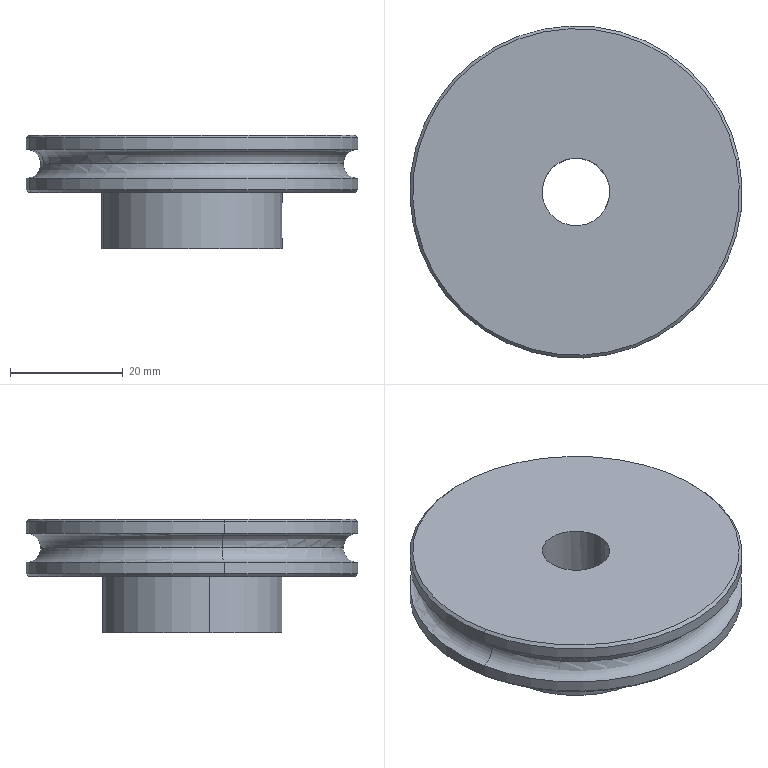Component | SolidWorks | TAR-02-031LargePulley-1 | 1 solid | 21 faces | box 59 x 59 x 20.19 mm | volume 31541 mm3 | cylinder 10 | torus 4 | cone 4 | plane 3 | commonest cylinder face diameters 59 x4 4.2 x2 12 x2 32 x2
build123d program:
from build123d import *

# Parameters (mm, degrees)
SKETCH2_R             = 16
BOSS_EXTRUDE1_DEPTH   = 10
SKETCH3_R             = 6
CUT_EXTRUDE1_DEPTH    = 36
M5_TAPPED_HOLE1_D     = 4.2
M5_TAPPED_HOLE1_DEPTH = 12.4
M5_TAPPED_HOLE1_TIP   = 1.262


with BuildPart() as part:
    # Sketch1 → Revolve1 (revolve)
    with BuildSketch(Plane.XY, mode=Mode.PRIVATE) as revolve1_sk:
        with BuildLine():
            Line((-30.231, 12.507), (-30.231, -16.493))
            Line((-30.231, -16.493), (-20.04, -16.493))
            Line((-20.04, -16.493), (-20.04, 12.507))
            Line((-20.04, 12.507), (-20.54, 13.007))
            Line((-20.54, 13.007), (-22.536, 13.007))
            ThreePointArc((-22.536, 13.007), (-25.136, 10.407), (-27.736, 13.007))
            Line((-27.736, 13.007), (-29.731, 13.007))
            Line((-29.731, 13.007), (-30.231, 12.507))
        make_face()
    revolve(revolve1_sk.sketch.rotate(Axis((-30.231, -16.493, 0), (1, 0, 0)), 90), axis=Axis((-30.231, -16.493, 0), (1, 0, 0)))

    # Sketch2 → Boss-Extrude1 (add)
    with BuildSketch(Plane(origin=(-20.04, 0, 0), x_dir=(0, 0, -1), z_dir=(1, 0, 0))):
        with Locations(Location((0, -16.493, 0), (0, 0, 180))):
            Circle(SKETCH2_R)
    extrude(amount=BOSS_EXTRUDE1_DEPTH)

    # Sketch3 → Cut-Extrude1 (cut)
    with BuildSketch(Plane(origin=(-10.04, 0, 0), x_dir=(0, 0, -1), z_dir=(1, 0, 0))):
        with Locations((0, -16.493)):
            Circle(SKETCH3_R)
    extrude(amount=-CUT_EXTRUDE1_DEPTH, mode=Mode.SUBTRACT)

    # M5 Tapped Hole1
    with Locations(Plane(origin=(-15.04, -16.493, 16), x_dir=(1, 0, 0), z_dir=(0, 0, 1))):
        with Locations((0, 0)):
            Hole(M5_TAPPED_HOLE1_D / 2, depth=M5_TAPPED_HOLE1_DEPTH)
            with Locations((0, 0, -(M5_TAPPED_HOLE1_DEPTH + M5_TAPPED_HOLE1_TIP / 2))):  # 118° drill point
                Cone(0, M5_TAPPED_HOLE1_D / 2, M5_TAPPED_HOLE1_TIP, mode=Mode.SUBTRACT)


solid = part.part

# Placed as in the assembly
solid = solid.moved(Location((11.338, 25.453, -47.696), (-90, 78.561, 90)))
STEP:
#1=CARTESIAN_POINT('',(1.714,0.596,-0.7858));
#2=VERTEX_POINT('',#1);
#3=CARTESIAN_POINT('',(1.613,0.5757,-0.8882));
#4=VERTEX_POINT('',#3);
#5=CARTESIAN_POINT('',(1.714,0.596,-0.8882));
#6=DIRECTION('',(0.1983,-0.9801,0.));
#7=DIRECTION('',(0.9801,0.1983,0.));
#8=AXIS2_PLACEMENT_3D('',#5,#6,#7);
#9=CIRCLE('',#8,0.1024);
#10=EDGE_CURVE('',#2,#4,#9,.T.);
#11=ORIENTED_EDGE('',*,*,#10,.T.);
#12=CARTESIAN_POINT('',(-0.4629,0.1556,-0.8882));
#13=VERTEX_POINT('',#12);
#14=CARTESIAN_POINT('',(0.5752,0.3657,-0.8882));
#15=DIRECTION('',(0.,0.,1.));
#16=DIRECTION('',(1.,0.,0.));
#17=AXIS2_PLACEMENT_3D('',#14,#15,#16);
#18=CIRCLE('',#17,1.059);
#19=EDGE_CURVE('',#4,#13,#18,.T.);
#20=ORIENTED_EDGE('',*,*,#19,.T.);
#21=CARTESIAN_POINT('',(-0.5632,0.1353,-0.7858));
#22=VERTEX_POINT('',#21);
#23=CARTESIAN_POINT('',(-0.5632,0.1353,-0.8882));
#24=DIRECTION('',(-0.1983,0.9801,0.));
#25=DIRECTION('',(-0.9801,-0.1983,0.));
#26=AXIS2_PLACEMENT_3D('',#23,#24,#25);
#27=CIRCLE('',#26,0.1024);
#28=EDGE_CURVE('',#22,#13,#27,.T.);
#29=ORIENTED_EDGE('',*,*,#28,.F.);
#30=CARTESIAN_POINT('',(0.5752,0.3657,-0.7858));
#31=DIRECTION('',(0.,0.,1.));
#32=DIRECTION('',(0.9801,0.1983,0.));
#33=AXIS2_PLACEMENT_3D('',#30,#31,#32);
#34=CIRCLE('',#33,1.161);
#35=EDGE_CURVE('',#2,#22,#34,.T.);
#36=ORIENTED_EDGE('',*,*,#35,.F.);
#37=EDGE_LOOP('',(#11,#20,#29,#36));
#38=FACE_OUTER_BOUND('',#37,.T.);
#39=CARTESIAN_POINT('',(0.5752,0.3657,-0.8882));
#40=DIRECTION('',(0.,0.,1.));
#41=DIRECTION('',(0.9801,0.1983,0.));
#42=AXIS2_PLACEMENT_3D('',#39,#40,#41);
#43=TOROIDAL_SURFACE('',#42,1.161,0.1024);
#44=ADVANCED_FACE('',(#38),#43,.F.);
#45=ORIENTED_EDGE('',*,*,#28,.T.);
#46=CARTESIAN_POINT('',(0.5752,0.3657,-0.8882));
#47=DIRECTION('',(0.,0.,1.));
#48=DIRECTION('',(1.,0.,0.));
#49=AXIS2_PLACEMENT_3D('',#46,#47,#48);
#50=CIRCLE('',#49,1.059);
#51=EDGE_CURVE('',#13,#4,#50,.T.);
#52=ORIENTED_EDGE('',*,*,#51,.T.);
#53=ORIENTED_EDGE('',*,*,#10,.F.);
#54=CARTESIAN_POINT('',(0.5752,0.3657,-0.7858));
#55=DIRECTION('',(0.,0.,1.));
#56=DIRECTION('',(0.9801,0.1983,0.));
#57=AXIS2_PLACEMENT_3D('',#54,#55,#56);
#58=CIRCLE('',#57,1.161);
#59=EDGE_CURVE('',#22,#2,#58,.T.);
#60=ORIENTED_EDGE('',*,*,#59,.F.);
#61=EDGE_LOOP('',(#45,#52,#53,#60));
#62=FACE_OUTER_BOUND('',#61,.T.);
#63=CARTESIAN_POINT('',(0.5752,0.3657,-0.8882));
#64=DIRECTION('',(0.,0.,1.));
#65=DIRECTION('',(0.9801,0.1983,0.));
#66=AXIS2_PLACEMENT_3D('',#63,#64,#65);
#67=TOROIDAL_SURFACE('',#66,1.161,0.1024);
#68=ADVANCED_FACE('',(#62),#67,.F.);
#69=CARTESIAN_POINT('',(0.8067,0.4125,-1.203));
#70=VERTEX_POINT('',#69);
#71=CARTESIAN_POINT('',(0.8067,0.4125,-1.368));
#72=VERTEX_POINT('',#71);
#73=CARTESIAN_POINT('',(0.8067,0.4125,-1.203));
#74=CARTESIAN_POINT('',(0.8078,0.4072,-1.203));
#75=CARTESIAN_POINT('',(0.8087,0.4018,-1.204));
#76=CARTESIAN_POINT('',(0.8101,0.3911,-1.206));
#77=CARTESIAN_POINT('',(0.8106,0.386,-1.207));
#78=CARTESIAN_POINT('',(0.8112,0.3759,-1.211));
#79=CARTESIAN_POINT('',(0.8114,0.371,-1.214));
#80=CARTESIAN_POINT('',(0.8114,0.3619,-1.22));
#81=CARTESIAN_POINT('',(0.8113,0.3577,-1.223));
#82=CARTESIAN_POINT('',(0.8107,0.3459,-1.235));
#83=CARTESIAN_POINT('',(0.81,0.3395,-1.244));
#84=CARTESIAN_POINT('',(0.8091,0.333,-1.259));
#85=CARTESIAN_POINT('',(0.8089,0.3313,-1.264));
#86=CARTESIAN_POINT('',(0.8085,0.3291,-1.275));
#87=CARTESIAN_POINT('',(0.8084,0.3285,-1.28));
#88=CARTESIAN_POINT('',(0.8084,0.3285,-1.291));
#89=CARTESIAN_POINT('',(0.8085,0.3291,-1.297));
#90=CARTESIAN_POINT('',(0.8089,0.3313,-1.307));
#91=CARTESIAN_POINT('',(0.8091,0.333,-1.312));
#92=CARTESIAN_POINT('',(0.81,0.3395,-1.327));
#93=CARTESIAN_POINT('',(0.8107,0.3459,-1.337));
#94=CARTESIAN_POINT('',(0.8113,0.3577,-1.348));
#95=CARTESIAN_POINT('',(0.8114,0.362,-1.351));
#96=CARTESIAN_POINT('',(0.8114,0.3711,-1.357));
#97=CARTESIAN_POINT('',(0.8112,0.3759,-1.36));
#98=CARTESIAN_POINT('',(0.8106,0.386,-1.364));
#99=CARTESIAN_POINT('',(0.8101,0.3912,-1.366));
#100=CARTESIAN_POINT('',(0.8087,0.4018,-1.368));
#101=CARTESIAN_POINT('',(0.8078,0.4071,-1.368));
#102=CARTESIAN_POINT('',(0.8067,0.4125,-1.368));
#103=B_SPLINE_CURVE_WITH_KNOTS('',3,(#73,#74,#75,#76,#77,#78,#79,#80,#81,#82,#83,#84,#85,#86,#87,#88,#89,#90,#91,#92,#93,#94,#95,#96,#97,#98,#99,#100,#101,#102),.UNSPECIFIED.,.F.,.F.,(4,2,2,2,2,2,2,2,2,2,2,2,2,2,4),(0.006618,0.007032,0.007445,0.007859,0.008273,0.0091,0.009513,0.009927,0.01034,0.01075,0.01158,0.01199,0.01241,0.01282,0.01324),.UNSPECIFIED.);
#104=EDGE_CURVE('',#70,#72,#103,.T.);
#105=ORIENTED_EDGE('',*,*,#104,.F.);
#106=CARTESIAN_POINT('',(1.193,0.4906,-1.203));
#107=VERTEX_POINT('',#106);
#108=CARTESIAN_POINT('',(1.193,0.4906,-1.203));
#109=DIRECTION('',(0.9801,0.1983,0.));
#110=VECTOR('',#109,39.37);
#111=LINE('',#108,#110);
#112=EDGE_CURVE('',#70,#107,#111,.T.);
#113=ORIENTED_EDGE('',*,*,#112,.T.);
#114=CARTESIAN_POINT('',(1.193,0.4906,-1.368));
#115=VERTEX_POINT('',#114);
#116=CARTESIAN_POINT('',(1.193,0.4906,-1.368));
#117=CARTESIAN_POINT('',(1.194,0.4852,-1.368));
#118=CARTESIAN_POINT('',(1.195,0.4799,-1.368));
#119=CARTESIAN_POINT('',(1.196,0.4695,-1.366));
#120=CARTESIAN_POINT('',(1.197,0.4643,-1.364));
#121=CARTESIAN_POINT('',(1.199,0.4544,-1.36));
#122=CARTESIAN_POINT('',(1.199,0.4497,-1.357));
#123=CARTESIAN_POINT('',(1.201,0.4408,-1.351));
#124=CARTESIAN_POINT('',(1.201,0.4365,-1.348));
#125=CARTESIAN_POINT('',(1.202,0.4251,-1.336));
#126=CARTESIAN_POINT('',(1.203,0.419,-1.327));
#127=CARTESIAN_POINT('',(1.203,0.4107,-1.307));
#128=CARTESIAN_POINT('',(1.204,0.4085,-1.296));
#129=CARTESIAN_POINT('',(1.204,0.4085,-1.28));
#130=CARTESIAN_POINT('',(1.204,0.409,-1.275));
#131=CARTESIAN_POINT('',(1.203,0.4111,-1.264));
#132=CARTESIAN_POINT('',(1.203,0.4127,-1.259));
#133=CARTESIAN_POINT('',(1.203,0.4169,-1.249));
#134=CARTESIAN_POINT('',(1.203,0.4195,-1.244));
#135=CARTESIAN_POINT('',(1.202,0.4255,-1.235));
#136=CARTESIAN_POINT('',(1.202,0.4289,-1.231));
#137=CARTESIAN_POINT('',(1.201,0.4366,-1.223));
#138=CARTESIAN_POINT('',(1.201,0.4407,-1.22));
#139=CARTESIAN_POINT('',(1.199,0.4497,-1.214));
#140=CARTESIAN_POINT('',(1.199,0.4545,-1.211));
#141=CARTESIAN_POINT('',(1.197,0.4644,-1.207));
#142=CARTESIAN_POINT('',(1.196,0.4695,-1.206));
#143=CARTESIAN_POINT('',(1.195,0.4799,-1.204));
#144=CARTESIAN_POINT('',(1.194,0.4853,-1.203));
#145=CARTESIAN_POINT('',(1.193,0.4906,-1.203));
#146=B_SPLINE_CURVE_WITH_KNOTS('',3,(#116,#117,#118,#119,#120,#121,#122,#123,#124,#125,#126,#127,#128,#129,#130,#131,#132,#133,#134,#135,#136,#137,#138,#139,#140,#141,#142,#143,#144,#145),.UNSPECIFIED.,.F.,.F.,(4,2,2,2,2,2,2,2,2,2,2,2,2,2,4),(0.,0.0004108,0.0008216,0.001232,0.001643,0.002465,0.003286,0.003697,0.004108,0.004519,0.004929,0.00534,0.005751,0.006162,0.006573),.UNSPECIFIED.);
#147=EDGE_CURVE('',#115,#107,#146,.T.);
#148=ORIENTED_EDGE('',*,*,#147,.F.);
#149=CARTESIAN_POINT('',(1.193,0.4906,-1.368));
#150=DIRECTION('',(0.9801,0.1983,0.));
#151=VECTOR('',#150,39.37);
#152=LINE('',#149,#151);
#153=EDGE_CURVE('',#72,#115,#152,.T.);
#154=ORIENTED_EDGE('',*,*,#153,.F.);
#155=EDGE_LOOP('',(#105,#113,#148,#154));
#156=FACE_OUTER_BOUND('',#155,.T.);
#157=CARTESIAN_POINT('',(1.193,0.4906,-1.286));
#158=DIRECTION('',(0.9801,0.1983,0.));
#159=DIRECTION('',(0.,0.,-1.));
#160=AXIS2_PLACEMENT_3D('',#157,#158,#159);
#161=CYLINDRICAL_SURFACE('',#160,0.08268);
#162=ADVANCED_FACE('',(#156),#161,.F.);
#163=CARTESIAN_POINT('',(0.8067,0.4125,-0.6876));
#164=VERTEX_POINT('',#163);
#165=CARTESIAN_POINT('',(0.3436,0.3188,-0.6876));
#166=VERTEX_POINT('',#165);
#167=CARTESIAN_POINT('',(0.5752,0.3657,-0.6876));
#168=DIRECTION('',(0.,0.,-1.));
#169=DIRECTION('',(-0.9801,-0.1983,0.));
#170=AXIS2_PLACEMENT_3D('',#167,#168,#169);
#171=CIRCLE('',#170,0.2362);
#172=EDGE_CURVE('',#164,#166,#171,.T.);
#173=ORIENTED_EDGE('',*,*,#172,.F.);
#174=CARTESIAN_POINT('',(0.8067,0.4125,-0.06517));
#175=DIRECTION('',(0.,0.,-1.));
#176=VECTOR('',#175,39.37);
#177=LINE('',#174,#176);
#178=EDGE_CURVE('',#164,#70,#177,.T.);
#179=ORIENTED_EDGE('',*,*,#178,.T.);
#180=ORIENTED_EDGE('',*,*,#104,.T.);
#181=CARTESIAN_POINT('',(0.8067,0.4125,-1.482));
#182=VERTEX_POINT('',#181);
#183=CARTESIAN_POINT('',(0.8067,0.4125,-0.06517));
#184=DIRECTION('',(0.,0.,-1.));
#185=VECTOR('',#184,39.37);
#186=LINE('',#183,#185);
#187=EDGE_CURVE('',#72,#182,#186,.T.);
#188=ORIENTED_EDGE('',*,*,#187,.T.);
#189=CARTESIAN_POINT('',(0.3436,0.3188,-1.482));
#190=VERTEX_POINT('',#189);
#191=CARTESIAN_POINT('',(0.5752,0.3657,-1.482));
#192=DIRECTION('',(0.,0.,-1.));
#193=DIRECTION('',(-0.9801,-0.1983,0.));
#194=AXIS2_PLACEMENT_3D('',#191,#192,#193);
#195=CIRCLE('',#194,0.2362);
#196=EDGE_CURVE('',#182,#190,#195,.T.);
#197=ORIENTED_EDGE('',*,*,#196,.T.);
#198=CARTESIAN_POINT('',(0.3436,0.3188,-0.06517));
#199=DIRECTION('',(0.,0.,-1.));
#200=VECTOR('',#199,39.37);
#201=LINE('',#198,#200);
#202=EDGE_CURVE('',#166,#190,#201,.T.);
#203=ORIENTED_EDGE('',*,*,#202,.F.);
#204=EDGE_LOOP('',(#173,#179,#180,#188,#197,#203));
#205=FACE_OUTER_BOUND('',#204,.T.);
#206=CARTESIAN_POINT('',(0.5752,0.3657,-0.06517));
#207=DIRECTION('',(0.,0.,-1.));
#208=DIRECTION('',(-0.9801,-0.1983,0.));
#209=AXIS2_PLACEMENT_3D('',#206,#207,#208);
#210=CYLINDRICAL_SURFACE('',#209,0.2362);
#211=ADVANCED_FACE('',(#205),#210,.F.);
#212=CARTESIAN_POINT('',(-0.04225,0.2407,-1.482));
#213=VERTEX_POINT('',#212);
#214=CARTESIAN_POINT('',(1.193,0.4906,-1.482));
#215=VERTEX_POINT('',#214);
#216=CARTESIAN_POINT('',(0.5752,0.3657,-1.482));
#217=DIRECTION('',(0.,0.,-1.));
#218=DIRECTION('',(-0.9801,-0.1983,0.));
#219=AXIS2_PLACEMENT_3D('',#216,#217,#218);
#220=CIRCLE('',#219,0.6299);
#221=EDGE_CURVE('',#213,#215,#220,.T.);
#222=ORIENTED_EDGE('',*,*,#221,.F.);
#223=CARTESIAN_POINT('',(-0.04225,0.2407,-1.089));
#224=VERTEX_POINT('',#223);
#225=CARTESIAN_POINT('',(-0.04225,0.2407,-1.482));
#226=DIRECTION('',(0.,0.,1.));
#227=VECTOR('',#226,39.37);
#228=LINE('',#225,#227);
#229=EDGE_CURVE('',#213,#224,#228,.T.);
#230=ORIENTED_EDGE('',*,*,#229,.T.);
#231=CARTESIAN_POINT('',(1.193,0.4906,-1.089));
#232=VERTEX_POINT('',#231);
#233=CARTESIAN_POINT('',(0.5752,0.3657,-1.089));
#234=DIRECTION('',(0.,0.,-1.));
#235=DIRECTION('',(0.9801,0.1983,0.));
#236=AXIS2_PLACEMENT_3D('',#233,#234,#235);
#237=CIRCLE('',#236,0.6299);
#238=EDGE_CURVE('',#224,#232,#237,.T.);
#239=ORIENTED_EDGE('',*,*,#238,.T.);
#240=CARTESIAN_POINT('',(1.193,0.4906,-1.482));
#241=DIRECTION('',(0.,0.,1.));
#242=VECTOR('',#241,39.37);
#243=LINE('',#240,#242);
#244=EDGE_CURVE('',#107,#232,#243,.T.);
#245=ORIENTED_EDGE('',*,*,#244,.F.);
#246=CARTESIAN_POINT('',(1.193,0.4906,-1.203));
#247=CARTESIAN_POINT('',(1.19,0.5012,-1.203));
#248=CARTESIAN_POINT('',(1.188,0.5118,-1.205));
#249=CARTESIAN_POINT('',(1.183,0.5311,-1.213));
#250=CARTESIAN_POINT('',(1.181,0.54,-1.22));
#251=CARTESIAN_POINT('',(1.177,0.551,-1.231));
#252=CARTESIAN_POINT('',(1.176,0.5543,-1.235));
#253=CARTESIAN_POINT('',(1.174,0.5601,-1.244));
#254=CARTESIAN_POINT('',(1.174,0.5625,-1.249));
#255=CARTESIAN_POINT('',(1.172,0.5665,-1.259));
#256=CARTESIAN_POINT('',(1.172,0.568,-1.264));
#257=CARTESIAN_POINT('',(1.171,0.57,-1.275));
#258=CARTESIAN_POINT('',(1.171,0.5705,-1.28));
#259=CARTESIAN_POINT('',(1.171,0.5705,-1.291));
#260=CARTESIAN_POINT('',(1.171,0.57,-1.296));
#261=CARTESIAN_POINT('',(1.172,0.568,-1.307));
#262=CARTESIAN_POINT('',(1.172,0.5665,-1.312));
#263=CARTESIAN_POINT('',(1.174,0.5626,-1.322));
#264=CARTESIAN_POINT('',(1.174,0.5601,-1.327));
#265=CARTESIAN_POINT('',(1.176,0.5544,-1.336));
#266=CARTESIAN_POINT('',(1.177,0.551,-1.34));
#267=CARTESIAN_POINT('',(1.181,0.5401,-1.352));
#268=CARTESIAN_POINT('',(1.183,0.5312,-1.358));
#269=CARTESIAN_POINT('',(1.188,0.5119,-1.366));
#270=CARTESIAN_POINT('',(1.19,0.5013,-1.368));
#271=CARTESIAN_POINT('',(1.193,0.4906,-1.368));
#272=B_SPLINE_CURVE_WITH_KNOTS('',3,(#246,#247,#248,#249,#250,#251,#252,#253,#254,#255,#256,#257,#258,#259,#260,#261,#262,#263,#264,#265,#266,#267,#268,#269,#270,#271),.UNSPECIFIED.,.F.,.F.,(4,2,2,2,2,2,2,2,2,2,2,2,4),(0.006573,0.007394,0.008215,0.008626,0.009037,0.009447,0.009858,0.01027,0.01068,0.01109,0.0115,0.01232,0.01314),.UNSPECIFIED.);
#273=EDGE_CURVE('',#107,#115,#272,.T.);
#274=ORIENTED_EDGE('',*,*,#273,.T.);
#275=CARTESIAN_POINT('',(1.193,0.4906,-1.482));
#276=DIRECTION('',(0.,0.,1.));
#277=VECTOR('',#276,39.37);
#278=LINE('',#275,#277);
#279=EDGE_CURVE('',#215,#115,#278,.T.);
#280=ORIENTED_EDGE('',*,*,#279,.F.);
#281=EDGE_LOOP('',(#222,#230,#239,#245,#274,#280));
#282=FACE_OUTER_BOUND('',#281,.T.);
#283=CARTESIAN_POINT('',(0.5752,0.3657,-1.482));
#284=DIRECTION('',(0.,0.,1.));
#285=DIRECTION('',(0.9801,0.1983,0.));
#286=AXIS2_PLACEMENT_3D('',#283,#284,#285);
#287=CYLINDRICAL_SURFACE('',#286,0.6299);
#288=ADVANCED_FACE('',(#282),#287,.T.);
#289=CARTESIAN_POINT('',(1.694,0.5921,-0.6876));
#290=VERTEX_POINT('',#289);
#291=CARTESIAN_POINT('',(-0.5439,0.1392,-0.6876));
#292=VERTEX_POINT('',#291);
#293=CARTESIAN_POINT('',(0.5752,0.3657,-0.6876));
#294=DIRECTION('',(0.,0.,1.));
#295=DIRECTION('',(0.9801,0.1983,0.));
#296=AXIS2_PLACEMENT_3D('',#293,#294,#295);
#297=CIRCLE('',#296,1.142);
#298=EDGE_CURVE('',#290,#292,#297,.T.);
#299=ORIENTED_EDGE('',*,*,#298,.F.);
#300=CARTESIAN_POINT('',(1.714,0.596,-0.7073));
#301=VERTEX_POINT('',#300);
#302=CARTESIAN_POINT('',(1.714,0.596,-0.7073));
#303=DIRECTION('',(0.6931,0.1402,-0.7071));
#304=VECTOR('',#303,39.37);
#305=LINE('',#302,#304);
#306=EDGE_CURVE('',#290,#301,#305,.T.);
#307=ORIENTED_EDGE('',*,*,#306,.T.);
#308=CARTESIAN_POINT('',(-0.5632,0.1353,-0.7073));
#309=VERTEX_POINT('',#308);
#310=CARTESIAN_POINT('',(0.5752,0.3657,-0.7073));
#311=DIRECTION('',(0.,0.,1.));
#312=DIRECTION('',(0.9801,0.1983,0.));
#313=AXIS2_PLACEMENT_3D('',#310,#311,#312);
#314=CIRCLE('',#313,1.161);
#315=EDGE_CURVE('',#301,#309,#314,.T.);
#316=ORIENTED_EDGE('',*,*,#315,.T.);
#317=CARTESIAN_POINT('',(-0.5632,0.1353,-0.7073));
#318=DIRECTION('',(-0.6931,-0.1402,-0.7071));
#319=VECTOR('',#318,39.37);
#320=LINE('',#317,#319);
#321=EDGE_CURVE('',#292,#309,#320,.T.);
#322=ORIENTED_EDGE('',*,*,#321,.F.);
#323=EDGE_LOOP('',(#299,#307,#316,#322));
#324=FACE_OUTER_BOUND('',#323,.T.);
#325=CARTESIAN_POINT('',(0.5752,0.3657,-0.7073));
#326=DIRECTION('',(0.,0.,-1.));
#327=DIRECTION('',(-0.9801,-0.1983,0.));
#328=AXIS2_PLACEMENT_3D('',#325,#326,#327);
#329=CONICAL_SURFACE('',#328,1.161,0.7854);
#330=ADVANCED_FACE('',(#324),#329,.T.);
#331=ORIENTED_EDGE('',*,*,#35,.T.);
#332=CARTESIAN_POINT('',(-0.5632,0.1353,-0.6876));
#333=DIRECTION('',(0.,0.,1.));
#334=VECTOR('',#333,39.37);
#335=LINE('',#332,#334);
#336=EDGE_CURVE('',#22,#309,#335,.T.);
#337=ORIENTED_EDGE('',*,*,#336,.T.);
#338=ORIENTED_EDGE('',*,*,#315,.F.);
#339=CARTESIAN_POINT('',(1.714,0.596,-0.6876));
#340=DIRECTION('',(0.,0.,1.));
#341=VECTOR('',#340,39.37);
#342=LINE('',#339,#341);
#343=EDGE_CURVE('',#2,#301,#342,.T.);
#344=ORIENTED_EDGE('',*,*,#343,.F.);
#345=EDGE_LOOP('',(#331,#337,#338,#344));
#346=FACE_OUTER_BOUND('',#345,.T.);
#347=CARTESIAN_POINT('',(0.5752,0.3657,-0.6876));
#348=DIRECTION('',(0.,0.,1.));
#349=DIRECTION('',(0.9801,0.1983,0.));
#350=AXIS2_PLACEMENT_3D('',#347,#348,#349);
#351=CYLINDRICAL_SURFACE('',#350,1.161);
#352=ADVANCED_FACE('',(#346),#351,.T.);
#353=ORIENTED_EDGE('',*,*,#51,.F.);
#354=CARTESIAN_POINT('',(-0.5632,0.1353,-0.9905));
#355=VERTEX_POINT('',#354);
#356=CARTESIAN_POINT('',(-0.5632,0.1353,-0.8882));
#357=DIRECTION('',(-0.1983,0.9801,0.));
#358=DIRECTION('',(-0.9801,-0.1983,0.));
#359=AXIS2_PLACEMENT_3D('',#356,#357,#358);
#360=CIRCLE('',#359,0.1024);
#361=EDGE_CURVE('',#13,#355,#360,.T.);
#362=ORIENTED_EDGE('',*,*,#361,.T.);
#363=CARTESIAN_POINT('',(1.714,0.596,-0.9905));
#364=VERTEX_POINT('',#363);
#365=CARTESIAN_POINT('',(0.5752,0.3657,-0.9905));
#366=DIRECTION('',(0.,0.,1.));
#367=DIRECTION('',(0.9801,0.1983,0.));
#368=AXIS2_PLACEMENT_3D('',#365,#366,#367);
#369=CIRCLE('',#368,1.161);
#370=EDGE_CURVE('',#355,#364,#369,.T.);
#371=ORIENTED_EDGE('',*,*,#370,.T.);
#372=CARTESIAN_POINT('',(1.714,0.596,-0.8882));
#373=DIRECTION('',(0.1983,-0.9801,0.));
#374=DIRECTION('',(0.9801,0.1983,0.));
#375=AXIS2_PLACEMENT_3D('',#372,#373,#374);
#376=CIRCLE('',#375,0.1024);
#377=EDGE_CURVE('',#4,#364,#376,.T.);
#378=ORIENTED_EDGE('',*,*,#377,.F.);
#379=EDGE_LOOP('',(#353,#362,#371,#378));
#380=FACE_OUTER_BOUND('',#379,.T.);
#381=CARTESIAN_POINT('',(0.5752,0.3657,-0.8882));
#382=DIRECTION('',(0.,0.,1.));
#383=DIRECTION('',(0.9801,0.1983,0.));
#384=AXIS2_PLACEMENT_3D('',#381,#382,#383);
#385=TOROIDAL_SURFACE('',#384,1.161,0.1024);
#386=ADVANCED_FACE('',(#380),#385,.F.);
#387=CARTESIAN_POINT('',(1.714,0.596,-1.069));
#388=VERTEX_POINT('',#387);
#389=CARTESIAN_POINT('',(-0.5632,0.1353,-1.069));
#390=VERTEX_POINT('',#389);
#391=CARTESIAN_POINT('',(0.5752,0.3657,-1.069));
#392=DIRECTION('',(0.,0.,1.));
#393=DIRECTION('',(0.9801,0.1983,0.));
#394=AXIS2_PLACEMENT_3D('',#391,#392,#393);
#395=CIRCLE('',#394,1.161);
#396=EDGE_CURVE('',#388,#390,#395,.T.);
#397=ORIENTED_EDGE('',*,*,#396,.T.);
#398=CARTESIAN_POINT('',(-0.5632,0.1353,-0.6876));
#399=DIRECTION('',(0.,0.,1.));
#400=VECTOR('',#399,39.37);
#401=LINE('',#398,#400);
#402=EDGE_CURVE('',#390,#355,#401,.T.);
#403=ORIENTED_EDGE('',*,*,#402,.T.);
#404=CARTESIAN_POINT('',(0.5752,0.3657,-0.9905));
#405=DIRECTION('',(0.,0.,1.));
#406=DIRECTION('',(0.9801,0.1983,0.));
#407=AXIS2_PLACEMENT_3D('',#404,#405,#406);
#408=CIRCLE('',#407,1.161);
#409=EDGE_CURVE('',#364,#355,#408,.T.);
#410=ORIENTED_EDGE('',*,*,#409,.F.);
#411=CARTESIAN_POINT('',(1.714,0.596,-0.6876));
#412=DIRECTION('',(0.,0.,1.));
#413=VECTOR('',#412,39.37);
#414=LINE('',#411,#413);
#415=EDGE_CURVE('',#388,#364,#414,.T.);
#416=ORIENTED_EDGE('',*,*,#415,.F.);
#417=EDGE_LOOP('',(#397,#403,#410,#416));
#418=FACE_OUTER_BOUND('',#417,.T.);
#419=CARTESIAN_POINT('',(0.5752,0.3657,-0.6876));
#420=DIRECTION('',(0.,0.,1.));
#421=DIRECTION('',(0.9801,0.1983,0.));
#422=AXIS2_PLACEMENT_3D('',#419,#420,#421);
#423=CYLINDRICAL_SURFACE('',#422,1.161);
#424=ADVANCED_FACE('',(#418),#423,.T.);
#425=CARTESIAN_POINT('',(1.694,0.5921,-1.089));
#426=VERTEX_POINT('',#425);
#427=CARTESIAN_POINT('',(-0.5439,0.1392,-1.089));
#428=VERTEX_POINT('',#427);
#429=CARTESIAN_POINT('',(0.5752,0.3657,-1.089));
#430=DIRECTION('',(0.,0.,1.));
#431=DIRECTION('',(0.9801,0.1983,0.));
#432=AXIS2_PLACEMENT_3D('',#429,#430,#431);
#433=CIRCLE('',#432,1.142);
#434=EDGE_CURVE('',#426,#428,#433,.T.);
#435=ORIENTED_EDGE('',*,*,#434,.T.);
#436=CARTESIAN_POINT('',(-0.5439,0.1392,-1.089));
#437=DIRECTION('',(-0.6931,-0.1402,0.7071));
#438=VECTOR('',#437,39.37);
#439=LINE('',#436,#438);
#440=EDGE_CURVE('',#428,#390,#439,.T.);
#441=ORIENTED_EDGE('',*,*,#440,.T.);
#442=ORIENTED_EDGE('',*,*,#396,.F.);
#443=CARTESIAN_POINT('',(1.694,0.5921,-1.089));
#444=DIRECTION('',(0.6931,0.1402,0.7071));
#445=VECTOR('',#444,39.37);
#446=LINE('',#443,#445);
#447=EDGE_CURVE('',#426,#388,#446,.T.);
#448=ORIENTED_EDGE('',*,*,#447,.F.);
#449=EDGE_LOOP('',(#435,#441,#442,#448));
#450=FACE_OUTER_BOUND('',#449,.T.);
#451=CARTESIAN_POINT('',(0.5752,0.3657,-1.089));
#452=DIRECTION('',(0.,0.,1.));
#453=DIRECTION('',(0.9801,0.1983,0.));
#454=AXIS2_PLACEMENT_3D('',#451,#452,#453);
#455=CONICAL_SURFACE('',#454,1.142,0.7854);
#456=ADVANCED_FACE('',(#450),#455,.T.);
#457=CARTESIAN_POINT('',(0.5752,0.3657,-1.089));
#458=DIRECTION('',(0.,0.,-1.));
#459=DIRECTION('',(0.9801,0.1983,0.));
#460=AXIS2_PLACEMENT_3D('',#457,#458,#459);
#461=CIRCLE('',#460,0.6299);
#462=EDGE_CURVE('',#232,#224,#461,.T.);
#463=ORIENTED_EDGE('',*,*,#462,.F.);
#464=ORIENTED_EDGE('',*,*,#238,.F.);
#465=EDGE_LOOP('',(#463,#464));
#466=FACE_BOUND('',#465,.T.);
#467=ORIENTED_EDGE('',*,*,#434,.F.);
#468=CARTESIAN_POINT('',(0.5752,0.3657,-1.089));
#469=DIRECTION('',(0.,0.,1.));
#470=DIRECTION('',(0.9801,0.1983,0.));
#471=AXIS2_PLACEMENT_3D('',#468,#469,#470);
#472=CIRCLE('',#471,1.142);
#473=EDGE_CURVE('',#428,#426,#472,.T.);
#474=ORIENTED_EDGE('',*,*,#473,.F.);
#475=EDGE_LOOP('',(#467,#474));
#476=FACE_OUTER_BOUND('',#475,.T.);
#477=CARTESIAN_POINT('',(0.5752,0.3657,-1.089));
#478=DIRECTION('',(0.,0.,1.));
#479=DIRECTION('',(0.9801,0.1983,0.));
#480=AXIS2_PLACEMENT_3D('',#477,#478,#479);
#481=PLANE('',#480);
#482=ADVANCED_FACE('',(#466,#476),#481,.F.);
#483=ORIENTED_EDGE('',*,*,#440,.F.);
#484=ORIENTED_EDGE('',*,*,#473,.T.);
#485=ORIENTED_EDGE('',*,*,#447,.T.);
#486=CARTESIAN_POINT('',(0.5752,0.3657,-1.069));
#487=DIRECTION('',(0.,0.,1.));
#488=DIRECTION('',(0.9801,0.1983,0.));
#489=AXIS2_PLACEMENT_3D('',#486,#487,#488);
#490=CIRCLE('',#489,1.161);
#491=EDGE_CURVE('',#390,#388,#490,.T.);
#492=ORIENTED_EDGE('',*,*,#491,.F.);
#493=EDGE_LOOP('',(#483,#484,#485,#492));
#494=FACE_OUTER_BOUND('',#493,.T.);
#495=CARTESIAN_POINT('',(0.5752,0.3657,-1.089));
#496=DIRECTION('',(0.,0.,1.));
#497=DIRECTION('',(0.9801,0.1983,0.));
#498=AXIS2_PLACEMENT_3D('',#495,#496,#497);
#499=CONICAL_SURFACE('',#498,1.142,0.7854);
#500=ADVANCED_FACE('',(#494),#499,.T.);
#501=ORIENTED_EDGE('',*,*,#402,.F.);
#502=ORIENTED_EDGE('',*,*,#491,.T.);
#503=ORIENTED_EDGE('',*,*,#415,.T.);
#504=ORIENTED_EDGE('',*,*,#370,.F.);
#505=EDGE_LOOP('',(#501,#502,#503,#504));
#506=FACE_OUTER_BOUND('',#505,.T.);
#507=CARTESIAN_POINT('',(0.5752,0.3657,-0.6876));
#508=DIRECTION('',(0.,0.,1.));
#509=DIRECTION('',(0.9801,0.1983,0.));
#510=AXIS2_PLACEMENT_3D('',#507,#508,#509);
#511=CYLINDRICAL_SURFACE('',#510,1.161);
#512=ADVANCED_FACE('',(#506),#511,.T.);
#513=ORIENTED_EDGE('',*,*,#19,.F.);
#514=ORIENTED_EDGE('',*,*,#377,.T.);
#515=ORIENTED_EDGE('',*,*,#409,.T.);
#516=ORIENTED_EDGE('',*,*,#361,.F.);
#517=EDGE_LOOP('',(#513,#514,#515,#516));
#518=FACE_OUTER_BOUND('',#517,.T.);
#519=CARTESIAN_POINT('',(0.5752,0.3657,-0.8882));
#520=DIRECTION('',(0.,0.,1.));
#521=DIRECTION('',(0.9801,0.1983,0.));
#522=AXIS2_PLACEMENT_3D('',#519,#520,#521);
#523=TOROIDAL_SURFACE('',#522,1.161,0.1024);
#524=ADVANCED_FACE('',(#518),#523,.F.);
#525=ORIENTED_EDGE('',*,*,#336,.F.);
#526=ORIENTED_EDGE('',*,*,#59,.T.);
#527=ORIENTED_EDGE('',*,*,#343,.T.);
#528=CARTESIAN_POINT('',(0.5752,0.3657,-0.7073));
#529=DIRECTION('',(0.,0.,1.));
#530=DIRECTION('',(0.9801,0.1983,0.));
#531=AXIS2_PLACEMENT_3D('',#528,#529,#530);
#532=CIRCLE('',#531,1.161);
#533=EDGE_CURVE('',#309,#301,#532,.T.);
#534=ORIENTED_EDGE('',*,*,#533,.F.);
#535=EDGE_LOOP('',(#525,#526,#527,#534));
#536=FACE_OUTER_BOUND('',#535,.T.);
#537=CARTESIAN_POINT('',(0.5752,0.3657,-0.6876));
#538=DIRECTION('',(0.,0.,1.));
#539=DIRECTION('',(0.9801,0.1983,0.));
#540=AXIS2_PLACEMENT_3D('',#537,#538,#539);
#541=CYLINDRICAL_SURFACE('',#540,1.161);
#542=ADVANCED_FACE('',(#536),#541,.T.);
#543=ORIENTED_EDGE('',*,*,#306,.F.);
#544=CARTESIAN_POINT('',(0.5752,0.3657,-0.6876));
#545=DIRECTION('',(0.,0.,1.));
#546=DIRECTION('',(0.9801,0.1983,0.));
#547=AXIS2_PLACEMENT_3D('',#544,#545,#546);
#548=CIRCLE('',#547,1.142);
#549=EDGE_CURVE('',#292,#290,#548,.T.);
#550=ORIENTED_EDGE('',*,*,#549,.F.);
#551=ORIENTED_EDGE('',*,*,#321,.T.);
#552=ORIENTED_EDGE('',*,*,#533,.T.);
#553=EDGE_LOOP('',(#543,#550,#551,#552));
#554=FACE_OUTER_BOUND('',#553,.T.);
#555=CARTESIAN_POINT('',(0.5752,0.3657,-0.7073));
#556=DIRECTION('',(0.,0.,-1.));
#557=DIRECTION('',(-0.9801,-0.1983,0.));
#558=AXIS2_PLACEMENT_3D('',#555,#556,#557);
#559=CONICAL_SURFACE('',#558,1.161,0.7854);
#560=ADVANCED_FACE('',(#554),#559,.T.);
#561=CARTESIAN_POINT('',(0.5752,0.3657,-0.6876));
#562=DIRECTION('',(0.,0.,-1.));
#563=DIRECTION('',(-0.9801,-0.1983,0.));
#564=AXIS2_PLACEMENT_3D('',#561,#562,#563);
#565=CIRCLE('',#564,0.2362);
#566=EDGE_CURVE('',#166,#164,#565,.T.);
#567=ORIENTED_EDGE('',*,*,#566,.T.);
#568=ORIENTED_EDGE('',*,*,#172,.T.);
#569=EDGE_LOOP('',(#567,#568));
#570=FACE_BOUND('',#569,.T.);
#571=ORIENTED_EDGE('',*,*,#549,.T.);
#572=ORIENTED_EDGE('',*,*,#298,.T.);
#573=EDGE_LOOP('',(#571,#572));
#574=FACE_OUTER_BOUND('',#573,.T.);
#575=CARTESIAN_POINT('',(0.3487,1.485,-0.6876));
#576=DIRECTION('',(0.,0.,-1.));
#577=DIRECTION('',(-0.9801,-0.1983,0.));
#578=AXIS2_PLACEMENT_3D('',#575,#576,#577);
#579=PLANE('',#578);
#580=ADVANCED_FACE('',(#570,#574),#579,.F.);
#581=ORIENTED_EDGE('',*,*,#229,.F.);
#582=CARTESIAN_POINT('',(0.5752,0.3657,-1.482));
#583=DIRECTION('',(0.,0.,-1.));
#584=DIRECTION('',(-0.9801,-0.1983,0.));
#585=AXIS2_PLACEMENT_3D('',#582,#583,#584);
#586=CIRCLE('',#585,0.6299);
#587=EDGE_CURVE('',#215,#213,#586,.T.);
#588=ORIENTED_EDGE('',*,*,#587,.F.);
#589=ORIENTED_EDGE('',*,*,#279,.T.);
#590=ORIENTED_EDGE('',*,*,#147,.T.);
#591=ORIENTED_EDGE('',*,*,#244,.T.);
#592=ORIENTED_EDGE('',*,*,#462,.T.);
#593=EDGE_LOOP('',(#581,#588,#589,#590,#591,#592));
#594=FACE_OUTER_BOUND('',#593,.T.);
#595=CARTESIAN_POINT('',(0.5752,0.3657,-1.482));
#596=DIRECTION('',(0.,0.,1.));
#597=DIRECTION('',(0.9801,0.1983,0.));
#598=AXIS2_PLACEMENT_3D('',#595,#596,#597);
#599=CYLINDRICAL_SURFACE('',#598,0.6299);
#600=ADVANCED_FACE('',(#594),#599,.T.);
#601=CARTESIAN_POINT('',(0.5752,0.3657,-1.482));
#602=DIRECTION('',(0.,0.,-1.));
#603=DIRECTION('',(-0.9801,-0.1983,0.));
#604=AXIS2_PLACEMENT_3D('',#601,#602,#603);
#605=CIRCLE('',#604,0.2362);
#606=EDGE_CURVE('',#190,#182,#605,.T.);
#607=ORIENTED_EDGE('',*,*,#606,.F.);
#608=ORIENTED_EDGE('',*,*,#196,.F.);
#609=EDGE_LOOP('',(#607,#608));
#610=FACE_BOUND('',#609,.T.);
#611=ORIENTED_EDGE('',*,*,#587,.T.);
#612=ORIENTED_EDGE('',*,*,#221,.T.);
#613=EDGE_LOOP('',(#611,#612));
#614=FACE_OUTER_BOUND('',#613,.T.);
#615=CARTESIAN_POINT('',(0.5752,0.3657,-1.482));
#616=DIRECTION('',(0.,0.,-1.));
#617=DIRECTION('',(-0.9801,-0.1983,0.));
#618=AXIS2_PLACEMENT_3D('',#615,#616,#617);
#619=PLANE('',#618);
#620=ADVANCED_FACE('',(#610,#614),#619,.T.);
#621=ORIENTED_EDGE('',*,*,#178,.F.);
#622=ORIENTED_EDGE('',*,*,#566,.F.);
#623=ORIENTED_EDGE('',*,*,#202,.T.);
#624=ORIENTED_EDGE('',*,*,#606,.T.);
#625=ORIENTED_EDGE('',*,*,#187,.F.);
#626=CARTESIAN_POINT('',(0.8067,0.4125,-1.368));
#627=CARTESIAN_POINT('',(0.8056,0.4179,-1.368));
#628=CARTESIAN_POINT('',(0.8043,0.4232,-1.368));
#629=CARTESIAN_POINT('',(0.8015,0.4334,-1.366));
#630=CARTESIAN_POINT('',(0.7999,0.4385,-1.364));
#631=CARTESIAN_POINT('',(0.7966,0.448,-1.36));
#632=CARTESIAN_POINT('',(0.7949,0.4525,-1.357));
#633=CARTESIAN_POINT('',(0.7914,0.4609,-1.351));
#634=CARTESIAN_POINT('',(0.7896,0.4649,-1.348));
#635=CARTESIAN_POINT('',(0.7845,0.4754,-1.337));
#636=CARTESIAN_POINT('',(0.7813,0.481,-1.327));
#637=CARTESIAN_POINT('',(0.778,0.4867,-1.312));
#638=CARTESIAN_POINT('',(0.7771,0.4881,-1.307));
#639=CARTESIAN_POINT('',(0.776,0.4901,-1.297));
#640=CARTESIAN_POINT('',(0.7756,0.4906,-1.291));
#641=CARTESIAN_POINT('',(0.7756,0.4906,-1.28));
#642=CARTESIAN_POINT('',(0.776,0.4901,-1.275));
#643=CARTESIAN_POINT('',(0.7771,0.4881,-1.264));
#644=CARTESIAN_POINT('',(0.778,0.4867,-1.259));
#645=CARTESIAN_POINT('',(0.7802,0.4829,-1.249));
#646=CARTESIAN_POINT('',(0.7816,0.4805,-1.244));
#647=CARTESIAN_POINT('',(0.7845,0.4751,-1.235));
#648=CARTESIAN_POINT('',(0.7862,0.4719,-1.231));
#649=CARTESIAN_POINT('',(0.7896,0.4648,-1.223));
#650=CARTESIAN_POINT('',(0.7914,0.4609,-1.22));
#651=CARTESIAN_POINT('',(0.7949,0.4525,-1.214));
#652=CARTESIAN_POINT('',(0.7966,0.448,-1.211));
#653=CARTESIAN_POINT('',(0.7999,0.4385,-1.207));
#654=CARTESIAN_POINT('',(0.8015,0.4335,-1.206));
#655=CARTESIAN_POINT('',(0.8043,0.4232,-1.204));
#656=CARTESIAN_POINT('',(0.8056,0.4178,-1.203));
#657=CARTESIAN_POINT('',(0.8067,0.4125,-1.203));
#658=B_SPLINE_CURVE_WITH_KNOTS('',3,(#626,#627,#628,#629,#630,#631,#632,#633,#634,#635,#636,#637,#638,#639,#640,#641,#642,#643,#644,#645,#646,#647,#648,#649,#650,#651,#652,#653,#654,#655,#656,#657),.UNSPECIFIED.,.F.,.F.,(4,2,2,2,2,2,2,2,2,2,2,2,2,2,2,4),(0.,0.0004136,0.0008273,0.001241,0.001655,0.002482,0.002896,0.003309,0.003723,0.004136,0.00455,0.004964,0.005377,0.005791,0.006205,0.006618),.UNSPECIFIED.);
#659=EDGE_CURVE('',#72,#70,#658,.T.);
#660=ORIENTED_EDGE('',*,*,#659,.T.);
#661=EDGE_LOOP('',(#621,#622,#623,#624,#625,#660));
#662=FACE_OUTER_BOUND('',#661,.T.);
#663=CARTESIAN_POINT('',(0.5752,0.3657,-0.06517));
#664=DIRECTION('',(0.,0.,-1.));
#665=DIRECTION('',(-0.9801,-0.1983,0.));
#666=AXIS2_PLACEMENT_3D('',#663,#664,#665);
#667=CYLINDRICAL_SURFACE('',#666,0.2362);
#668=ADVANCED_FACE('',(#662),#667,.F.);
#669=ORIENTED_EDGE('',*,*,#112,.F.);
#670=ORIENTED_EDGE('',*,*,#659,.F.);
#671=ORIENTED_EDGE('',*,*,#153,.T.);
#672=ORIENTED_EDGE('',*,*,#273,.F.);
#673=EDGE_LOOP('',(#669,#670,#671,#672));
#674=FACE_OUTER_BOUND('',#673,.T.);
#675=CARTESIAN_POINT('',(1.193,0.4906,-1.286));
#676=DIRECTION('',(0.9801,0.1983,0.));
#677=DIRECTION('',(0.,0.,-1.));
#678=AXIS2_PLACEMENT_3D('',#675,#676,#677);
#679=CYLINDRICAL_SURFACE('',#678,0.08268);
#680=ADVANCED_FACE('',(#674),#679,.F.);
#681=CLOSED_SHELL('',(#44,#68,#162,#211,#288,#330,#352,#386,#424,#456,#482,#500,#512,#524,#542,#560,#580,#600,#620,#668,#680));
#682=MANIFOLD_SOLID_BREP('',#681);
#683=CARTESIAN_POINT('',(0.,0.,0.));
#684=DIRECTION('',(0.,0.,1.));
#685=DIRECTION('',(1.,0.,0.));
#686=AXIS2_PLACEMENT_3D('',#683,#684,#685);
#687=(LENGTH_UNIT()NAMED_UNIT(*)SI_UNIT($,.METRE.));
#688=LENGTH_MEASURE_WITH_UNIT(LENGTH_MEASURE(0.0254),#687);
#689=DIMENSIONAL_EXPONENTS(1.,0.,0.,0.,0.,0.,0.);
#690=(CONVERSION_BASED_UNIT('',#688)LENGTH_UNIT()NAMED_UNIT(#689));
#691=UNCERTAINTY_MEASURE_WITH_UNIT(LENGTH_MEASURE(0.00001),#690,'','');
#692=(NAMED_UNIT(*)PLANE_ANGLE_UNIT()SI_UNIT($,.RADIAN.));
#693=(NAMED_UNIT(*)SI_UNIT($,.STERADIAN.)SOLID_ANGLE_UNIT());
#694=(GEOMETRIC_REPRESENTATION_CONTEXT(3)GLOBAL_UNCERTAINTY_ASSIGNED_CONTEXT((#691))GLOBAL_UNIT_ASSIGNED_CONTEXT((#690,#692,#693))REPRESENTATION_CONTEXT('',''));
#695=ADVANCED_BREP_SHAPE_REPRESENTATION('',(#682,#686),#694);
#696=COLOUR_RGB('',0.7922,0.8196,0.9333);
#697=FILL_AREA_STYLE_COLOUR('',#696);
#698=FILL_AREA_STYLE('',(#697));
#699=SURFACE_STYLE_FILL_AREA(#698);
#700=SURFACE_SIDE_STYLE('',(#699));
#701=SURFACE_STYLE_USAGE(.BOTH.,#700);
#702=PRESENTATION_STYLE_ASSIGNMENT((#701));
#703=STYLED_ITEM('',(#702),#682);
#704=(LENGTH_UNIT()NAMED_UNIT(*)SI_UNIT($,.METRE.));
#705=LENGTH_MEASURE_WITH_UNIT(LENGTH_MEASURE(0.0254),#704);
#706=DIMENSIONAL_EXPONENTS(1.,0.,0.,0.,0.,0.,0.);
#707=(CONVERSION_BASED_UNIT('',#705)LENGTH_UNIT()NAMED_UNIT(#706));
#708=UNCERTAINTY_MEASURE_WITH_UNIT(LENGTH_MEASURE(0.00001),#707,'','');
#709=(NAMED_UNIT(*)PLANE_ANGLE_UNIT()SI_UNIT($,.RADIAN.));
#710=(NAMED_UNIT(*)SI_UNIT($,.STERADIAN.)SOLID_ANGLE_UNIT());
#711=(GEOMETRIC_REPRESENTATION_CONTEXT(3)GLOBAL_UNCERTAINTY_ASSIGNED_CONTEXT((#708))GLOBAL_UNIT_ASSIGNED_CONTEXT((#707,#709,#710))REPRESENTATION_CONTEXT('',''));
#712=MECHANICAL_DESIGN_GEOMETRIC_PRESENTATION_REPRESENTATION('',(#703),#711);
#713=PRESENTATION_LAYER_ASSIGNMENT('','',(#703));